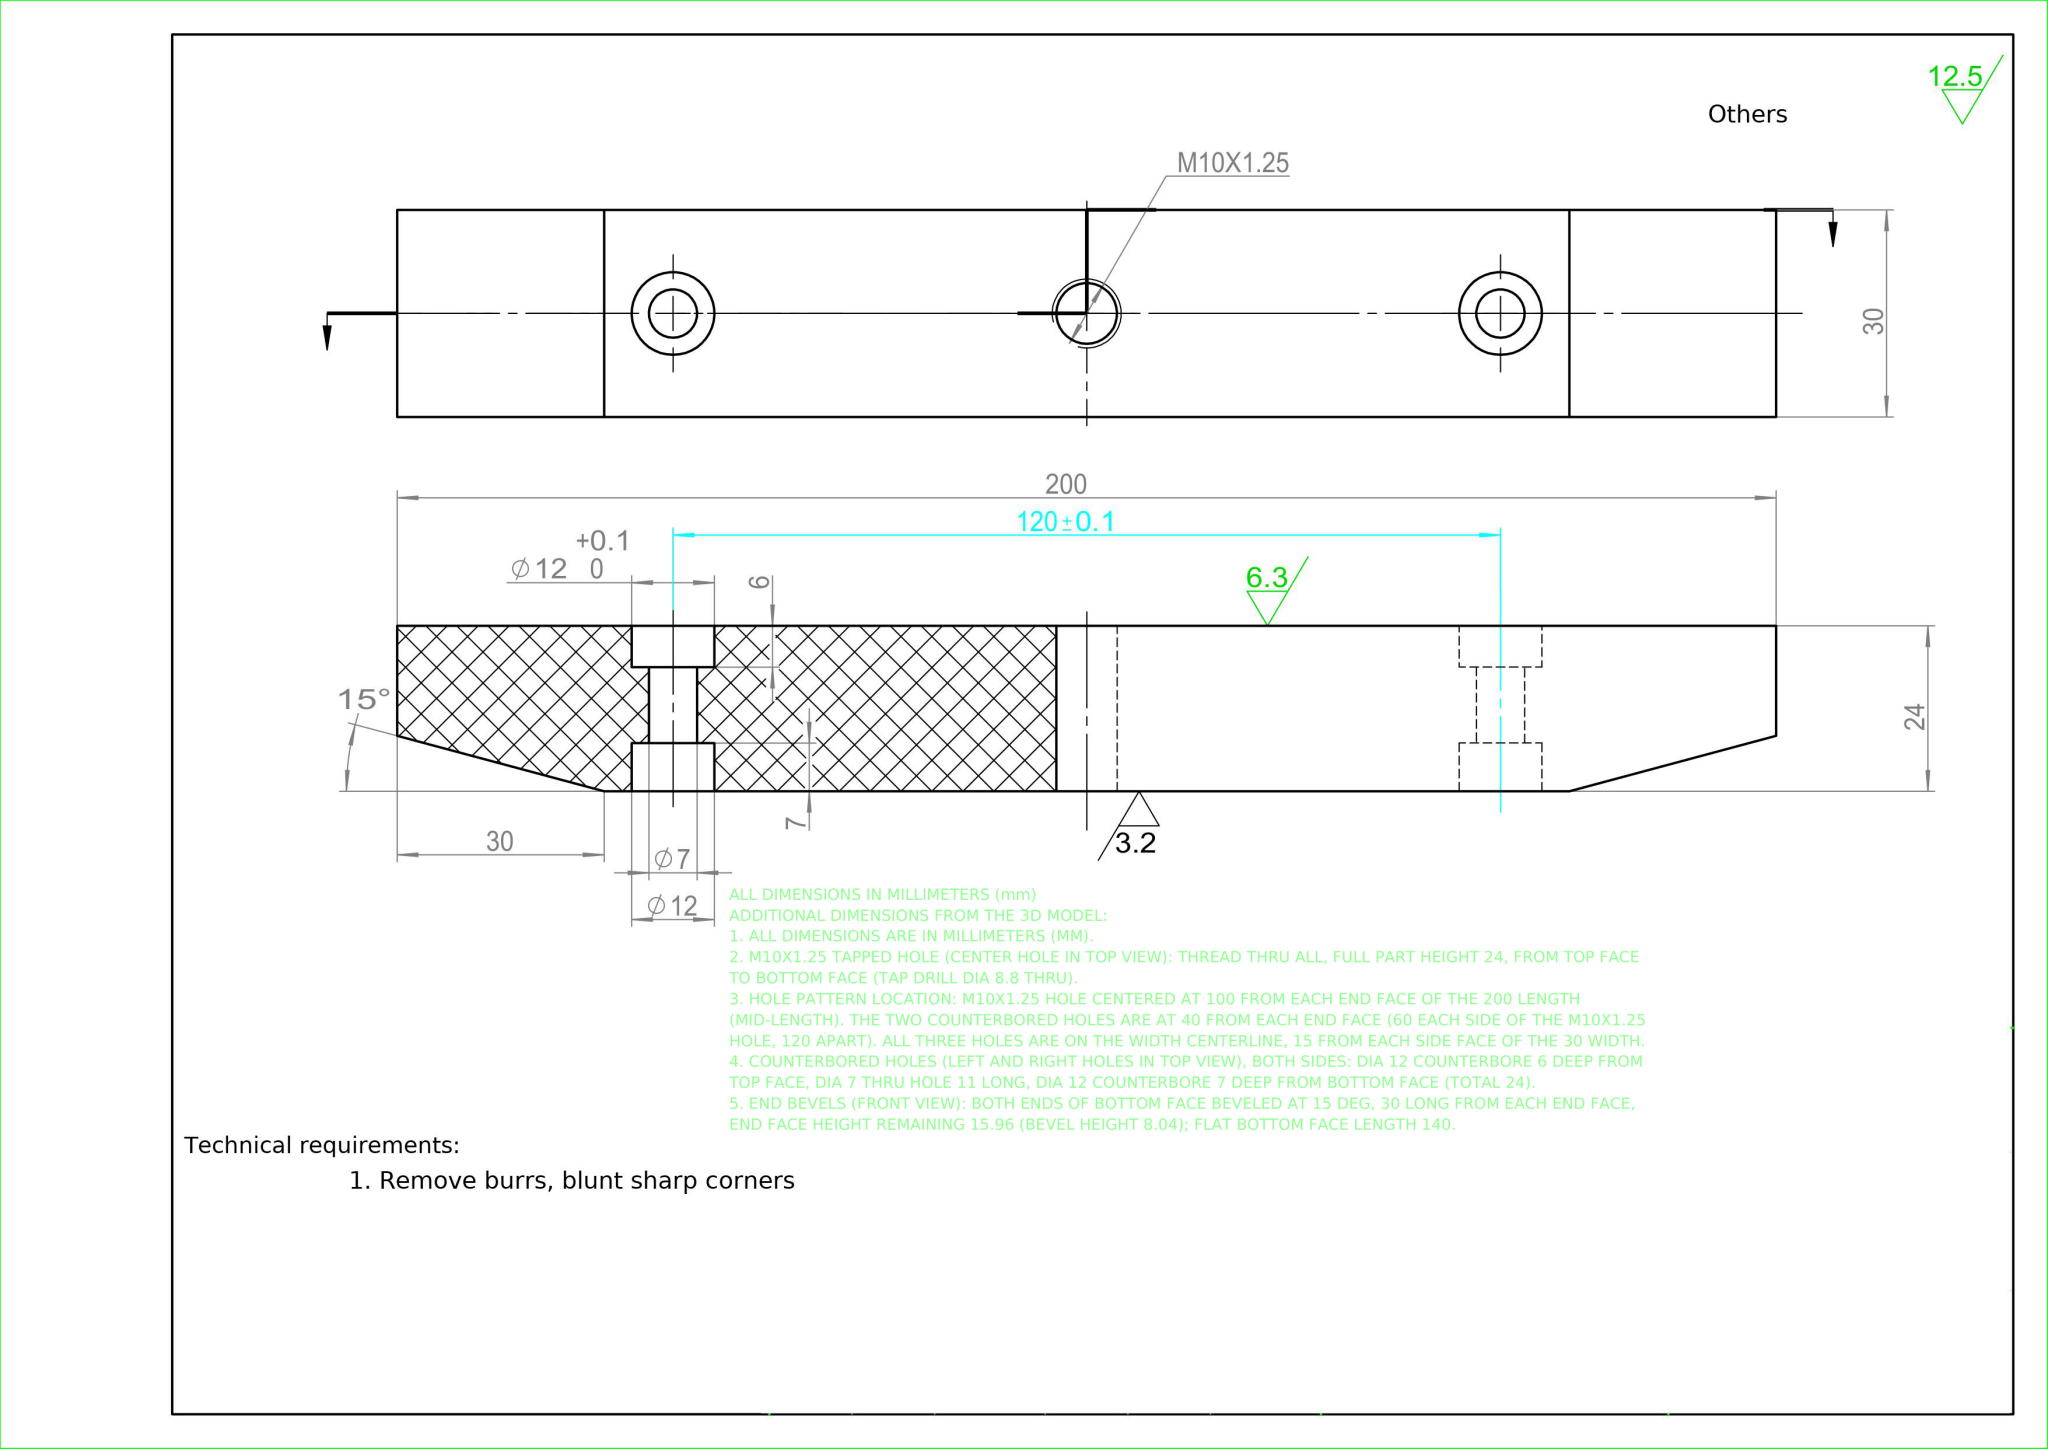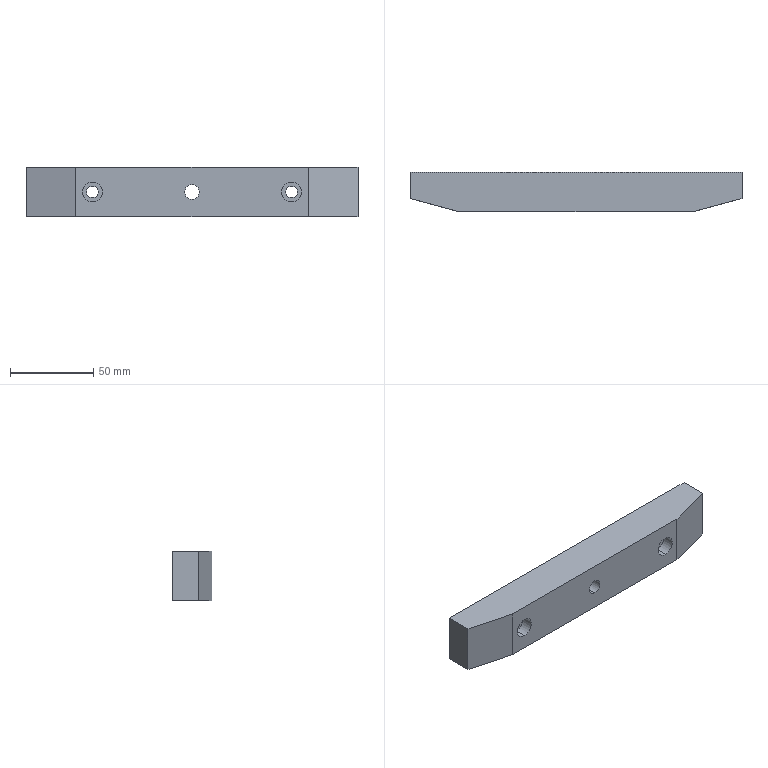Part | NX | mm | Tapered Threaded Mounting Bar | 1 solid | 26 faces | box 200 x 24 x 30 mm | volume 131518 mm3 | cylinder 14 | plane 12 | commonest cylinder face diameters 12 x8 7 x4 8.8 x2
STEP:
#1=COLOUR_RGB('',1.,1.,0.);
#2=FILL_AREA_STYLE_COLOUR('',#1);
#3=FILL_AREA_STYLE('',(#2));
#4=SURFACE_STYLE_FILL_AREA(#3);
#5=SURFACE_SIDE_STYLE('',(#4));
#6=SURFACE_STYLE_USAGE(.BOTH.,#5);
#7=PRESENTATION_STYLE_ASSIGNMENT((#6));
#8=CARTESIAN_POINT('',(66.,18.,15.));
#9=VERTEX_POINT('',#8);
#10=CARTESIAN_POINT('',(54.,18.,15.));
#11=VERTEX_POINT('',#10);
#12=CARTESIAN_POINT('',(60.,18.,15.));
#13=DIRECTION('',(-0.,1.,0.));
#14=DIRECTION('',(-1.,0.,0.));
#15=AXIS2_PLACEMENT_3D('',#12,#13,#14);
#16=CIRCLE('',#15,6.);
#17=EDGE_CURVE('',#9,#11,#16,.T.);
#18=ORIENTED_EDGE('',*,*,#17,.F.);
#19=CARTESIAN_POINT('',(66.,24.,15.));
#20=VERTEX_POINT('',#19);
#21=CARTESIAN_POINT('',(66.,18.,15.));
#22=DIRECTION('',(-0.,1.,0.));
#23=VECTOR('',#22,1000.);
#24=LINE('',#21,#23);
#25=EDGE_CURVE('',#9,#20,#24,.T.);
#26=ORIENTED_EDGE('',*,*,#25,.T.);
#27=CARTESIAN_POINT('',(54.,24.,15.));
#28=VERTEX_POINT('',#27);
#29=CARTESIAN_POINT('',(60.,24.,15.));
#30=DIRECTION('',(-0.,1.,0.));
#31=DIRECTION('',(-1.,0.,0.));
#32=AXIS2_PLACEMENT_3D('',#29,#30,#31);
#33=CIRCLE('',#32,6.);
#34=EDGE_CURVE('',#20,#28,#33,.T.);
#35=ORIENTED_EDGE('',*,*,#34,.T.);
#36=CARTESIAN_POINT('',(54.,18.,15.));
#37=DIRECTION('',(-0.,1.,0.));
#38=VECTOR('',#37,1000.);
#39=LINE('',#36,#38);
#40=EDGE_CURVE('',#11,#28,#39,.T.);
#41=ORIENTED_EDGE('',*,*,#40,.F.);
#42=EDGE_LOOP('',(#18,#26,#35,#41));
#43=FACE_OUTER_BOUND('',#42,.T.);
#44=CARTESIAN_POINT('',(60.,18.,15.));
#45=DIRECTION('',(-0.,1.,0.));
#46=DIRECTION('',(-1.,0.,0.));
#47=AXIS2_PLACEMENT_3D('',#44,#45,#46);
#48=CYLINDRICAL_SURFACE('',#47,6.);
#49=ADVANCED_FACE('',(#43),#48,.F.);
#50=CARTESIAN_POINT('',(-54.,18.,15.));
#51=VERTEX_POINT('',#50);
#52=CARTESIAN_POINT('',(-66.,18.,15.));
#53=VERTEX_POINT('',#52);
#54=CARTESIAN_POINT('',(-60.,18.,15.));
#55=DIRECTION('',(-0.,1.,0.));
#56=DIRECTION('',(-1.,0.,0.));
#57=AXIS2_PLACEMENT_3D('',#54,#55,#56);
#58=CIRCLE('',#57,6.);
#59=EDGE_CURVE('',#51,#53,#58,.T.);
#60=ORIENTED_EDGE('',*,*,#59,.F.);
#61=CARTESIAN_POINT('',(-54.,24.,15.));
#62=VERTEX_POINT('',#61);
#63=CARTESIAN_POINT('',(-54.,18.,15.));
#64=DIRECTION('',(-0.,1.,0.));
#65=VECTOR('',#64,1000.);
#66=LINE('',#63,#65);
#67=EDGE_CURVE('',#51,#62,#66,.T.);
#68=ORIENTED_EDGE('',*,*,#67,.T.);
#69=CARTESIAN_POINT('',(-66.,24.,15.));
#70=VERTEX_POINT('',#69);
#71=CARTESIAN_POINT('',(-60.,24.,15.));
#72=DIRECTION('',(-0.,1.,0.));
#73=DIRECTION('',(-1.,0.,0.));
#74=AXIS2_PLACEMENT_3D('',#71,#72,#73);
#75=CIRCLE('',#74,6.);
#76=EDGE_CURVE('',#62,#70,#75,.T.);
#77=ORIENTED_EDGE('',*,*,#76,.T.);
#78=CARTESIAN_POINT('',(-66.,18.,15.));
#79=DIRECTION('',(-0.,1.,0.));
#80=VECTOR('',#79,1000.);
#81=LINE('',#78,#80);
#82=EDGE_CURVE('',#53,#70,#81,.T.);
#83=ORIENTED_EDGE('',*,*,#82,.F.);
#84=EDGE_LOOP('',(#60,#68,#77,#83));
#85=FACE_OUTER_BOUND('',#84,.T.);
#86=CARTESIAN_POINT('',(-60.,18.,15.));
#87=DIRECTION('',(-0.,1.,0.));
#88=DIRECTION('',(-1.,0.,0.));
#89=AXIS2_PLACEMENT_3D('',#86,#87,#88);
#90=CYLINDRICAL_SURFACE('',#89,6.);
#91=ADVANCED_FACE('',(#85),#90,.F.);
#92=CARTESIAN_POINT('',(-60.,7.,21.));
#93=VERTEX_POINT('',#92);
#94=CARTESIAN_POINT('',(-60.,7.,9.));
#95=VERTEX_POINT('',#94);
#96=CARTESIAN_POINT('',(-60.,7.,15.));
#97=DIRECTION('',(0.,-1.,0.));
#98=DIRECTION('',(0.,0.,-1.));
#99=AXIS2_PLACEMENT_3D('',#96,#97,#98);
#100=CIRCLE('',#99,6.);
#101=EDGE_CURVE('',#93,#95,#100,.T.);
#102=ORIENTED_EDGE('',*,*,#101,.F.);
#103=CARTESIAN_POINT('',(-60.,-0.,21.));
#104=VERTEX_POINT('',#103);
#105=CARTESIAN_POINT('',(-60.,-0.,21.));
#106=DIRECTION('',(0.,-1.,0.));
#107=VECTOR('',#106,1000.);
#108=LINE('',#105,#107);
#109=EDGE_CURVE('',#93,#104,#108,.T.);
#110=ORIENTED_EDGE('',*,*,#109,.T.);
#111=CARTESIAN_POINT('',(-60.,-0.,9.));
#112=VERTEX_POINT('',#111);
#113=CARTESIAN_POINT('',(-60.,-0.,15.));
#114=DIRECTION('',(0.,-1.,0.));
#115=DIRECTION('',(0.,0.,-1.));
#116=AXIS2_PLACEMENT_3D('',#113,#114,#115);
#117=CIRCLE('',#116,6.);
#118=EDGE_CURVE('',#104,#112,#117,.T.);
#119=ORIENTED_EDGE('',*,*,#118,.T.);
#120=CARTESIAN_POINT('',(-60.,-0.,9.));
#121=DIRECTION('',(0.,-1.,0.));
#122=VECTOR('',#121,1000.);
#123=LINE('',#120,#122);
#124=EDGE_CURVE('',#95,#112,#123,.T.);
#125=ORIENTED_EDGE('',*,*,#124,.F.);
#126=EDGE_LOOP('',(#102,#110,#119,#125));
#127=FACE_OUTER_BOUND('',#126,.T.);
#128=CARTESIAN_POINT('',(-60.,-0.,15.));
#129=DIRECTION('',(0.,-1.,0.));
#130=DIRECTION('',(0.,0.,-1.));
#131=AXIS2_PLACEMENT_3D('',#128,#129,#130);
#132=CYLINDRICAL_SURFACE('',#131,6.);
#133=ADVANCED_FACE('',(#127),#132,.F.);
#134=CARTESIAN_POINT('',(60.,7.,21.));
#135=VERTEX_POINT('',#134);
#136=CARTESIAN_POINT('',(60.,7.,9.));
#137=VERTEX_POINT('',#136);
#138=CARTESIAN_POINT('',(60.,7.,15.));
#139=DIRECTION('',(0.,-1.,0.));
#140=DIRECTION('',(0.,0.,-1.));
#141=AXIS2_PLACEMENT_3D('',#138,#139,#140);
#142=CIRCLE('',#141,6.);
#143=EDGE_CURVE('',#135,#137,#142,.T.);
#144=ORIENTED_EDGE('',*,*,#143,.F.);
#145=CARTESIAN_POINT('',(60.,0.,21.));
#146=VERTEX_POINT('',#145);
#147=CARTESIAN_POINT('',(60.,0.,21.));
#148=DIRECTION('',(0.,-1.,0.));
#149=VECTOR('',#148,1000.);
#150=LINE('',#147,#149);
#151=EDGE_CURVE('',#135,#146,#150,.T.);
#152=ORIENTED_EDGE('',*,*,#151,.T.);
#153=CARTESIAN_POINT('',(60.,0.,9.));
#154=VERTEX_POINT('',#153);
#155=CARTESIAN_POINT('',(60.,0.,15.));
#156=DIRECTION('',(0.,-1.,0.));
#157=DIRECTION('',(0.,0.,-1.));
#158=AXIS2_PLACEMENT_3D('',#155,#156,#157);
#159=CIRCLE('',#158,6.);
#160=EDGE_CURVE('',#146,#154,#159,.T.);
#161=ORIENTED_EDGE('',*,*,#160,.T.);
#162=CARTESIAN_POINT('',(60.,0.,9.));
#163=DIRECTION('',(0.,-1.,0.));
#164=VECTOR('',#163,1000.);
#165=LINE('',#162,#164);
#166=EDGE_CURVE('',#137,#154,#165,.T.);
#167=ORIENTED_EDGE('',*,*,#166,.F.);
#168=EDGE_LOOP('',(#144,#152,#161,#167));
#169=FACE_OUTER_BOUND('',#168,.T.);
#170=CARTESIAN_POINT('',(60.,0.,15.));
#171=DIRECTION('',(0.,-1.,0.));
#172=DIRECTION('',(0.,0.,-1.));
#173=AXIS2_PLACEMENT_3D('',#170,#171,#172);
#174=CYLINDRICAL_SURFACE('',#173,6.);
#175=ADVANCED_FACE('',(#169),#174,.F.);
#176=CARTESIAN_POINT('',(0.,24.,19.4));
#177=VERTEX_POINT('',#176);
#178=CARTESIAN_POINT('',(0.,24.,10.6));
#179=VERTEX_POINT('',#178);
#180=CARTESIAN_POINT('',(0.,24.,15.));
#181=DIRECTION('',(0.,-1.,0.));
#182=DIRECTION('',(0.,0.,-1.));
#183=AXIS2_PLACEMENT_3D('',#180,#181,#182);
#184=CIRCLE('',#183,4.4);
#185=EDGE_CURVE('',#177,#179,#184,.T.);
#186=ORIENTED_EDGE('',*,*,#185,.F.);
#187=CARTESIAN_POINT('',(0.,-0.,19.4));
#188=VERTEX_POINT('',#187);
#189=CARTESIAN_POINT('',(0.,0.,19.4));
#190=DIRECTION('',(0.,-1.,0.));
#191=VECTOR('',#190,1000.);
#192=LINE('',#189,#191);
#193=EDGE_CURVE('',#177,#188,#192,.T.);
#194=ORIENTED_EDGE('',*,*,#193,.T.);
#195=CARTESIAN_POINT('',(0.,-0.,10.6));
#196=VERTEX_POINT('',#195);
#197=CARTESIAN_POINT('',(0.,-0.,15.));
#198=DIRECTION('',(0.,-1.,0.));
#199=DIRECTION('',(0.,0.,-1.));
#200=AXIS2_PLACEMENT_3D('',#197,#198,#199);
#201=CIRCLE('',#200,4.4);
#202=EDGE_CURVE('',#188,#196,#201,.T.);
#203=ORIENTED_EDGE('',*,*,#202,.T.);
#204=CARTESIAN_POINT('',(0.,0.,10.6));
#205=DIRECTION('',(0.,-1.,0.));
#206=VECTOR('',#205,1000.);
#207=LINE('',#204,#206);
#208=EDGE_CURVE('',#179,#196,#207,.T.);
#209=ORIENTED_EDGE('',*,*,#208,.F.);
#210=EDGE_LOOP('',(#186,#194,#203,#209));
#211=FACE_OUTER_BOUND('',#210,.T.);
#212=CARTESIAN_POINT('',(0.,0.,15.));
#213=DIRECTION('',(0.,-1.,0.));
#214=DIRECTION('',(0.,0.,-1.));
#215=AXIS2_PLACEMENT_3D('',#212,#213,#214);
#216=CYLINDRICAL_SURFACE('',#215,4.4);
#217=ADVANCED_FACE('',(#211),#216,.F.);
#218=CARTESIAN_POINT('',(-60.,18.,18.5));
#219=VERTEX_POINT('',#218);
#220=CARTESIAN_POINT('',(-60.,18.,11.5));
#221=VERTEX_POINT('',#220);
#222=CARTESIAN_POINT('',(-60.,18.,15.));
#223=DIRECTION('',(0.,-1.,0.));
#224=DIRECTION('',(-1.,0.,0.));
#225=AXIS2_PLACEMENT_3D('',#222,#223,#224);
#226=CIRCLE('',#225,3.5);
#227=EDGE_CURVE('',#219,#221,#226,.T.);
#228=ORIENTED_EDGE('',*,*,#227,.F.);
#229=CARTESIAN_POINT('',(-60.,7.,18.5));
#230=VERTEX_POINT('',#229);
#231=CARTESIAN_POINT('',(-60.,-0.,18.5));
#232=DIRECTION('',(0.,-1.,0.));
#233=VECTOR('',#232,1000.);
#234=LINE('',#231,#233);
#235=EDGE_CURVE('',#219,#230,#234,.T.);
#236=ORIENTED_EDGE('',*,*,#235,.T.);
#237=CARTESIAN_POINT('',(-60.,7.,11.5));
#238=VERTEX_POINT('',#237);
#239=CARTESIAN_POINT('',(-60.,7.,15.));
#240=DIRECTION('',(0.,-1.,0.));
#241=DIRECTION('',(0.,0.,-1.));
#242=AXIS2_PLACEMENT_3D('',#239,#240,#241);
#243=CIRCLE('',#242,3.5);
#244=EDGE_CURVE('',#230,#238,#243,.T.);
#245=ORIENTED_EDGE('',*,*,#244,.T.);
#246=CARTESIAN_POINT('',(-60.,-0.,11.5));
#247=DIRECTION('',(0.,-1.,0.));
#248=VECTOR('',#247,1000.);
#249=LINE('',#246,#248);
#250=EDGE_CURVE('',#221,#238,#249,.T.);
#251=ORIENTED_EDGE('',*,*,#250,.F.);
#252=EDGE_LOOP('',(#228,#236,#245,#251));
#253=FACE_OUTER_BOUND('',#252,.T.);
#254=CARTESIAN_POINT('',(-60.,-0.,15.));
#255=DIRECTION('',(0.,-1.,0.));
#256=DIRECTION('',(0.,0.,-1.));
#257=AXIS2_PLACEMENT_3D('',#254,#255,#256);
#258=CYLINDRICAL_SURFACE('',#257,3.5);
#259=ADVANCED_FACE('',(#253),#258,.F.);
#260=CARTESIAN_POINT('',(60.,18.,18.5));
#261=VERTEX_POINT('',#260);
#262=CARTESIAN_POINT('',(60.,18.,11.5));
#263=VERTEX_POINT('',#262);
#264=CARTESIAN_POINT('',(60.,18.,15.));
#265=DIRECTION('',(0.,-1.,0.));
#266=DIRECTION('',(-1.,0.,0.));
#267=AXIS2_PLACEMENT_3D('',#264,#265,#266);
#268=CIRCLE('',#267,3.5);
#269=EDGE_CURVE('',#261,#263,#268,.T.);
#270=ORIENTED_EDGE('',*,*,#269,.F.);
#271=CARTESIAN_POINT('',(60.,7.,18.5));
#272=VERTEX_POINT('',#271);
#273=CARTESIAN_POINT('',(60.,0.,18.5));
#274=DIRECTION('',(0.,-1.,0.));
#275=VECTOR('',#274,1000.);
#276=LINE('',#273,#275);
#277=EDGE_CURVE('',#261,#272,#276,.T.);
#278=ORIENTED_EDGE('',*,*,#277,.T.);
#279=CARTESIAN_POINT('',(60.,7.,11.5));
#280=VERTEX_POINT('',#279);
#281=CARTESIAN_POINT('',(60.,7.,15.));
#282=DIRECTION('',(0.,-1.,0.));
#283=DIRECTION('',(0.,0.,-1.));
#284=AXIS2_PLACEMENT_3D('',#281,#282,#283);
#285=CIRCLE('',#284,3.5);
#286=EDGE_CURVE('',#272,#280,#285,.T.);
#287=ORIENTED_EDGE('',*,*,#286,.T.);
#288=CARTESIAN_POINT('',(60.,0.,11.5));
#289=DIRECTION('',(0.,-1.,0.));
#290=VECTOR('',#289,1000.);
#291=LINE('',#288,#290);
#292=EDGE_CURVE('',#263,#280,#291,.T.);
#293=ORIENTED_EDGE('',*,*,#292,.F.);
#294=EDGE_LOOP('',(#270,#278,#287,#293));
#295=FACE_OUTER_BOUND('',#294,.T.);
#296=CARTESIAN_POINT('',(60.,0.,15.));
#297=DIRECTION('',(0.,-1.,0.));
#298=DIRECTION('',(0.,0.,-1.));
#299=AXIS2_PLACEMENT_3D('',#296,#297,#298);
#300=CYLINDRICAL_SURFACE('',#299,3.5);
#301=ADVANCED_FACE('',(#295),#300,.F.);
#302=ORIENTED_EDGE('',*,*,#277,.F.);
#303=CARTESIAN_POINT('',(60.,18.,15.));
#304=DIRECTION('',(0.,-1.,0.));
#305=DIRECTION('',(-1.,0.,0.));
#306=AXIS2_PLACEMENT_3D('',#303,#304,#305);
#307=CIRCLE('',#306,3.5);
#308=EDGE_CURVE('',#263,#261,#307,.T.);
#309=ORIENTED_EDGE('',*,*,#308,.F.);
#310=ORIENTED_EDGE('',*,*,#292,.T.);
#311=CARTESIAN_POINT('',(60.,7.,15.));
#312=DIRECTION('',(0.,-1.,0.));
#313=DIRECTION('',(0.,0.,-1.));
#314=AXIS2_PLACEMENT_3D('',#311,#312,#313);
#315=CIRCLE('',#314,3.5);
#316=EDGE_CURVE('',#280,#272,#315,.T.);
#317=ORIENTED_EDGE('',*,*,#316,.T.);
#318=EDGE_LOOP('',(#302,#309,#310,#317));
#319=FACE_OUTER_BOUND('',#318,.T.);
#320=CARTESIAN_POINT('',(60.,0.,15.));
#321=DIRECTION('',(0.,-1.,0.));
#322=DIRECTION('',(0.,0.,-1.));
#323=AXIS2_PLACEMENT_3D('',#320,#321,#322);
#324=CYLINDRICAL_SURFACE('',#323,3.5);
#325=ADVANCED_FACE('',(#319),#324,.F.);
#326=ORIENTED_EDGE('',*,*,#235,.F.);
#327=CARTESIAN_POINT('',(-60.,18.,15.));
#328=DIRECTION('',(0.,-1.,0.));
#329=DIRECTION('',(-1.,0.,0.));
#330=AXIS2_PLACEMENT_3D('',#327,#328,#329);
#331=CIRCLE('',#330,3.5);
#332=EDGE_CURVE('',#221,#219,#331,.T.);
#333=ORIENTED_EDGE('',*,*,#332,.F.);
#334=ORIENTED_EDGE('',*,*,#250,.T.);
#335=CARTESIAN_POINT('',(-60.,7.,15.));
#336=DIRECTION('',(0.,-1.,0.));
#337=DIRECTION('',(0.,0.,-1.));
#338=AXIS2_PLACEMENT_3D('',#335,#336,#337);
#339=CIRCLE('',#338,3.5);
#340=EDGE_CURVE('',#238,#230,#339,.T.);
#341=ORIENTED_EDGE('',*,*,#340,.T.);
#342=EDGE_LOOP('',(#326,#333,#334,#341));
#343=FACE_OUTER_BOUND('',#342,.T.);
#344=CARTESIAN_POINT('',(-60.,-0.,15.));
#345=DIRECTION('',(0.,-1.,0.));
#346=DIRECTION('',(0.,0.,-1.));
#347=AXIS2_PLACEMENT_3D('',#344,#345,#346);
#348=CYLINDRICAL_SURFACE('',#347,3.5);
#349=ADVANCED_FACE('',(#343),#348,.F.);
#350=CARTESIAN_POINT('',(70.,-0.,0.));
#351=VERTEX_POINT('',#350);
#352=CARTESIAN_POINT('',(100.,8.038,0.));
#353=VERTEX_POINT('',#352);
#354=CARTESIAN_POINT('',(100.,8.038,0.));
#355=DIRECTION('',(0.9659,0.2588,0.));
#356=VECTOR('',#355,1000.);
#357=LINE('',#354,#356);
#358=EDGE_CURVE('',#351,#353,#357,.T.);
#359=ORIENTED_EDGE('',*,*,#358,.T.);
#360=CARTESIAN_POINT('',(100.,8.038,30.));
#361=VERTEX_POINT('',#360);
#362=CARTESIAN_POINT('',(100.,8.038,30.));
#363=DIRECTION('',(0.,0.,-1.));
#364=VECTOR('',#363,1000.);
#365=LINE('',#362,#364);
#366=EDGE_CURVE('',#361,#353,#365,.T.);
#367=ORIENTED_EDGE('',*,*,#366,.F.);
#368=CARTESIAN_POINT('',(70.,-0.,30.));
#369=VERTEX_POINT('',#368);
#370=CARTESIAN_POINT('',(100.,8.038,30.));
#371=DIRECTION('',(0.9659,0.2588,0.));
#372=VECTOR('',#371,1000.);
#373=LINE('',#370,#372);
#374=EDGE_CURVE('',#369,#361,#373,.T.);
#375=ORIENTED_EDGE('',*,*,#374,.F.);
#376=CARTESIAN_POINT('',(70.,-0.,30.));
#377=DIRECTION('',(0.,0.,-1.));
#378=VECTOR('',#377,1000.);
#379=LINE('',#376,#378);
#380=EDGE_CURVE('',#369,#351,#379,.T.);
#381=ORIENTED_EDGE('',*,*,#380,.T.);
#382=EDGE_LOOP('',(#359,#367,#375,#381));
#383=FACE_OUTER_BOUND('',#382,.T.);
#384=CARTESIAN_POINT('',(100.,8.038,30.));
#385=DIRECTION('',(-0.2588,0.9659,0.));
#386=DIRECTION('',(-0.9659,-0.2588,0.));
#387=AXIS2_PLACEMENT_3D('',#384,#385,#386);
#388=PLANE('',#387);
#389=ADVANCED_FACE('',(#383),#388,.F.);
#390=CARTESIAN_POINT('',(100.,24.,0.));
#391=VERTEX_POINT('',#390);
#392=CARTESIAN_POINT('',(100.,8.038,0.));
#393=DIRECTION('',(0.,1.,0.));
#394=VECTOR('',#393,1000.);
#395=LINE('',#392,#394);
#396=EDGE_CURVE('',#353,#391,#395,.T.);
#397=ORIENTED_EDGE('',*,*,#396,.T.);
#398=CARTESIAN_POINT('',(100.,24.,30.));
#399=VERTEX_POINT('',#398);
#400=CARTESIAN_POINT('',(100.,24.,30.));
#401=DIRECTION('',(0.,0.,-1.));
#402=VECTOR('',#401,1000.);
#403=LINE('',#400,#402);
#404=EDGE_CURVE('',#399,#391,#403,.T.);
#405=ORIENTED_EDGE('',*,*,#404,.F.);
#406=CARTESIAN_POINT('',(100.,8.038,30.));
#407=DIRECTION('',(0.,1.,0.));
#408=VECTOR('',#407,1000.);
#409=LINE('',#406,#408);
#410=EDGE_CURVE('',#361,#399,#409,.T.);
#411=ORIENTED_EDGE('',*,*,#410,.F.);
#412=ORIENTED_EDGE('',*,*,#366,.T.);
#413=EDGE_LOOP('',(#397,#405,#411,#412));
#414=FACE_OUTER_BOUND('',#413,.T.);
#415=CARTESIAN_POINT('',(100.,8.038,30.));
#416=DIRECTION('',(-1.,0.,0.));
#417=DIRECTION('',(0.,0.,1.));
#418=AXIS2_PLACEMENT_3D('',#415,#416,#417);
#419=PLANE('',#418);
#420=ADVANCED_FACE('',(#414),#419,.F.);
#421=CARTESIAN_POINT('',(60.,24.,15.));
#422=DIRECTION('',(-0.,1.,0.));
#423=DIRECTION('',(-1.,0.,0.));
#424=AXIS2_PLACEMENT_3D('',#421,#422,#423);
#425=CIRCLE('',#424,6.);
#426=EDGE_CURVE('',#28,#20,#425,.T.);
#427=ORIENTED_EDGE('',*,*,#426,.F.);
#428=ORIENTED_EDGE('',*,*,#34,.F.);
#429=EDGE_LOOP('',(#427,#428));
#430=FACE_BOUND('',#429,.T.);
#431=CARTESIAN_POINT('',(-60.,24.,15.));
#432=DIRECTION('',(-0.,1.,0.));
#433=DIRECTION('',(-1.,0.,0.));
#434=AXIS2_PLACEMENT_3D('',#431,#432,#433);
#435=CIRCLE('',#434,6.);
#436=EDGE_CURVE('',#70,#62,#435,.T.);
#437=ORIENTED_EDGE('',*,*,#436,.F.);
#438=ORIENTED_EDGE('',*,*,#76,.F.);
#439=EDGE_LOOP('',(#437,#438));
#440=FACE_BOUND('',#439,.T.);
#441=CARTESIAN_POINT('',(0.,24.,15.));
#442=DIRECTION('',(0.,-1.,0.));
#443=DIRECTION('',(0.,0.,-1.));
#444=AXIS2_PLACEMENT_3D('',#441,#442,#443);
#445=CIRCLE('',#444,4.4);
#446=EDGE_CURVE('',#179,#177,#445,.T.);
#447=ORIENTED_EDGE('',*,*,#446,.T.);
#448=ORIENTED_EDGE('',*,*,#185,.T.);
#449=EDGE_LOOP('',(#447,#448));
#450=FACE_BOUND('',#449,.T.);
#451=CARTESIAN_POINT('',(-100.,24.,0.));
#452=VERTEX_POINT('',#451);
#453=CARTESIAN_POINT('',(-100.,24.,0.));
#454=DIRECTION('',(-1.,-0.,0.));
#455=VECTOR('',#454,1000.);
#456=LINE('',#453,#455);
#457=EDGE_CURVE('',#391,#452,#456,.T.);
#458=ORIENTED_EDGE('',*,*,#457,.T.);
#459=CARTESIAN_POINT('',(-100.,24.,30.));
#460=VERTEX_POINT('',#459);
#461=CARTESIAN_POINT('',(-100.,24.,30.));
#462=DIRECTION('',(0.,0.,-1.));
#463=VECTOR('',#462,1000.);
#464=LINE('',#461,#463);
#465=EDGE_CURVE('',#460,#452,#464,.T.);
#466=ORIENTED_EDGE('',*,*,#465,.F.);
#467=CARTESIAN_POINT('',(-100.,24.,30.));
#468=DIRECTION('',(-1.,-0.,0.));
#469=VECTOR('',#468,1000.);
#470=LINE('',#467,#469);
#471=EDGE_CURVE('',#399,#460,#470,.T.);
#472=ORIENTED_EDGE('',*,*,#471,.F.);
#473=ORIENTED_EDGE('',*,*,#404,.T.);
#474=EDGE_LOOP('',(#458,#466,#472,#473));
#475=FACE_OUTER_BOUND('',#474,.T.);
#476=CARTESIAN_POINT('',(-100.,24.,30.));
#477=DIRECTION('',(0.,-1.,0.));
#478=DIRECTION('',(1.,0.,0.));
#479=AXIS2_PLACEMENT_3D('',#476,#477,#478);
#480=PLANE('',#479);
#481=ADVANCED_FACE('',(#430,#440,#450,#475),#480,.F.);
#482=CARTESIAN_POINT('',(-100.,8.038,0.));
#483=VERTEX_POINT('',#482);
#484=CARTESIAN_POINT('',(-100.,8.038,0.));
#485=DIRECTION('',(0.,-1.,0.));
#486=VECTOR('',#485,1000.);
#487=LINE('',#484,#486);
#488=EDGE_CURVE('',#452,#483,#487,.T.);
#489=ORIENTED_EDGE('',*,*,#488,.T.);
#490=CARTESIAN_POINT('',(-100.,8.038,30.));
#491=VERTEX_POINT('',#490);
#492=CARTESIAN_POINT('',(-100.,8.038,30.));
#493=DIRECTION('',(0.,0.,-1.));
#494=VECTOR('',#493,1000.);
#495=LINE('',#492,#494);
#496=EDGE_CURVE('',#491,#483,#495,.T.);
#497=ORIENTED_EDGE('',*,*,#496,.F.);
#498=CARTESIAN_POINT('',(-100.,8.038,30.));
#499=DIRECTION('',(0.,-1.,0.));
#500=VECTOR('',#499,1000.);
#501=LINE('',#498,#500);
#502=EDGE_CURVE('',#460,#491,#501,.T.);
#503=ORIENTED_EDGE('',*,*,#502,.F.);
#504=ORIENTED_EDGE('',*,*,#465,.T.);
#505=EDGE_LOOP('',(#489,#497,#503,#504));
#506=FACE_OUTER_BOUND('',#505,.T.);
#507=CARTESIAN_POINT('',(-100.,8.038,30.));
#508=DIRECTION('',(1.,0.,0.));
#509=DIRECTION('',(0.,0.,-1.));
#510=AXIS2_PLACEMENT_3D('',#507,#508,#509);
#511=PLANE('',#510);
#512=ADVANCED_FACE('',(#506),#511,.F.);
#513=CARTESIAN_POINT('',(-70.,-0.,0.));
#514=VERTEX_POINT('',#513);
#515=CARTESIAN_POINT('',(-100.,8.038,0.));
#516=DIRECTION('',(0.9659,-0.2588,0.));
#517=VECTOR('',#516,1000.);
#518=LINE('',#515,#517);
#519=EDGE_CURVE('',#483,#514,#518,.T.);
#520=ORIENTED_EDGE('',*,*,#519,.T.);
#521=CARTESIAN_POINT('',(-70.,-0.,30.));
#522=VERTEX_POINT('',#521);
#523=CARTESIAN_POINT('',(-70.,-0.,30.));
#524=DIRECTION('',(0.,0.,-1.));
#525=VECTOR('',#524,1000.);
#526=LINE('',#523,#525);
#527=EDGE_CURVE('',#522,#514,#526,.T.);
#528=ORIENTED_EDGE('',*,*,#527,.F.);
#529=CARTESIAN_POINT('',(-100.,8.038,30.));
#530=DIRECTION('',(0.9659,-0.2588,0.));
#531=VECTOR('',#530,1000.);
#532=LINE('',#529,#531);
#533=EDGE_CURVE('',#491,#522,#532,.T.);
#534=ORIENTED_EDGE('',*,*,#533,.F.);
#535=ORIENTED_EDGE('',*,*,#496,.T.);
#536=EDGE_LOOP('',(#520,#528,#534,#535));
#537=FACE_OUTER_BOUND('',#536,.T.);
#538=CARTESIAN_POINT('',(-100.,8.038,30.));
#539=DIRECTION('',(0.2588,0.9659,0.));
#540=DIRECTION('',(-0.9659,0.2588,0.));
#541=AXIS2_PLACEMENT_3D('',#538,#539,#540);
#542=PLANE('',#541);
#543=ADVANCED_FACE('',(#537),#542,.F.);
#544=CARTESIAN_POINT('',(-60.,-0.,15.));
#545=DIRECTION('',(0.,-1.,0.));
#546=DIRECTION('',(0.,0.,-1.));
#547=AXIS2_PLACEMENT_3D('',#544,#545,#546);
#548=CIRCLE('',#547,6.);
#549=EDGE_CURVE('',#112,#104,#548,.T.);
#550=ORIENTED_EDGE('',*,*,#549,.F.);
#551=ORIENTED_EDGE('',*,*,#118,.F.);
#552=EDGE_LOOP('',(#550,#551));
#553=FACE_BOUND('',#552,.T.);
#554=CARTESIAN_POINT('',(60.,0.,15.));
#555=DIRECTION('',(0.,-1.,0.));
#556=DIRECTION('',(0.,0.,-1.));
#557=AXIS2_PLACEMENT_3D('',#554,#555,#556);
#558=CIRCLE('',#557,6.);
#559=EDGE_CURVE('',#154,#146,#558,.T.);
#560=ORIENTED_EDGE('',*,*,#559,.F.);
#561=ORIENTED_EDGE('',*,*,#160,.F.);
#562=EDGE_LOOP('',(#560,#561));
#563=FACE_BOUND('',#562,.T.);
#564=CARTESIAN_POINT('',(0.,-0.,15.));
#565=DIRECTION('',(0.,-1.,0.));
#566=DIRECTION('',(0.,0.,-1.));
#567=AXIS2_PLACEMENT_3D('',#564,#565,#566);
#568=CIRCLE('',#567,4.4);
#569=EDGE_CURVE('',#196,#188,#568,.T.);
#570=ORIENTED_EDGE('',*,*,#569,.F.);
#571=ORIENTED_EDGE('',*,*,#202,.F.);
#572=EDGE_LOOP('',(#570,#571));
#573=FACE_BOUND('',#572,.T.);
#574=CARTESIAN_POINT('',(-70.,-0.,0.));
#575=DIRECTION('',(1.,0.,0.));
#576=VECTOR('',#575,1000.);
#577=LINE('',#574,#576);
#578=EDGE_CURVE('',#514,#351,#577,.T.);
#579=ORIENTED_EDGE('',*,*,#578,.T.);
#580=ORIENTED_EDGE('',*,*,#380,.F.);
#581=CARTESIAN_POINT('',(-70.,-0.,30.));
#582=DIRECTION('',(1.,0.,0.));
#583=VECTOR('',#582,1000.);
#584=LINE('',#581,#583);
#585=EDGE_CURVE('',#522,#369,#584,.T.);
#586=ORIENTED_EDGE('',*,*,#585,.F.);
#587=ORIENTED_EDGE('',*,*,#527,.T.);
#588=EDGE_LOOP('',(#579,#580,#586,#587));
#589=FACE_OUTER_BOUND('',#588,.T.);
#590=CARTESIAN_POINT('',(-70.,-0.,30.));
#591=DIRECTION('',(-0.,1.,0.));
#592=DIRECTION('',(-1.,-0.,0.));
#593=AXIS2_PLACEMENT_3D('',#590,#591,#592);
#594=PLANE('',#593);
#595=ADVANCED_FACE('',(#553,#563,#573,#589),#594,.F.);
#596=ORIENTED_EDGE('',*,*,#374,.T.);
#597=ORIENTED_EDGE('',*,*,#410,.T.);
#598=ORIENTED_EDGE('',*,*,#471,.T.);
#599=ORIENTED_EDGE('',*,*,#502,.T.);
#600=ORIENTED_EDGE('',*,*,#533,.T.);
#601=ORIENTED_EDGE('',*,*,#585,.T.);
#602=EDGE_LOOP('',(#596,#597,#598,#599,#600,#601));
#603=FACE_OUTER_BOUND('',#602,.T.);
#604=CARTESIAN_POINT('',(-100.,-45.551,30.));
#605=DIRECTION('',(0.,0.,-1.));
#606=DIRECTION('',(-1.,0.,0.));
#607=AXIS2_PLACEMENT_3D('',#604,#605,#606);
#608=PLANE('',#607);
#609=ADVANCED_FACE('',(#603),#608,.F.);
#610=ORIENTED_EDGE('',*,*,#358,.F.);
#611=ORIENTED_EDGE('',*,*,#578,.F.);
#612=ORIENTED_EDGE('',*,*,#519,.F.);
#613=ORIENTED_EDGE('',*,*,#488,.F.);
#614=ORIENTED_EDGE('',*,*,#457,.F.);
#615=ORIENTED_EDGE('',*,*,#396,.F.);
#616=EDGE_LOOP('',(#610,#611,#612,#613,#614,#615));
#617=FACE_OUTER_BOUND('',#616,.T.);
#618=CARTESIAN_POINT('',(-100.,-45.551,0.));
#619=DIRECTION('',(0.,0.,-1.));
#620=DIRECTION('',(-1.,0.,0.));
#621=AXIS2_PLACEMENT_3D('',#618,#619,#620);
#622=PLANE('',#621);
#623=ADVANCED_FACE('',(#617),#622,.T.);
#624=ORIENTED_EDGE('',*,*,#193,.F.);
#625=ORIENTED_EDGE('',*,*,#446,.F.);
#626=ORIENTED_EDGE('',*,*,#208,.T.);
#627=ORIENTED_EDGE('',*,*,#569,.T.);
#628=EDGE_LOOP('',(#624,#625,#626,#627));
#629=FACE_OUTER_BOUND('',#628,.T.);
#630=CARTESIAN_POINT('',(0.,0.,15.));
#631=DIRECTION('',(0.,-1.,0.));
#632=DIRECTION('',(0.,0.,-1.));
#633=AXIS2_PLACEMENT_3D('',#630,#631,#632);
#634=CYLINDRICAL_SURFACE('',#633,4.4);
#635=ADVANCED_FACE('',(#629),#634,.F.);
#636=ORIENTED_EDGE('',*,*,#316,.F.);
#637=ORIENTED_EDGE('',*,*,#286,.F.);
#638=EDGE_LOOP('',(#636,#637));
#639=FACE_BOUND('',#638,.T.);
#640=CARTESIAN_POINT('',(60.,7.,15.));
#641=DIRECTION('',(0.,-1.,0.));
#642=DIRECTION('',(0.,0.,-1.));
#643=AXIS2_PLACEMENT_3D('',#640,#641,#642);
#644=CIRCLE('',#643,6.);
#645=EDGE_CURVE('',#137,#135,#644,.T.);
#646=ORIENTED_EDGE('',*,*,#645,.T.);
#647=ORIENTED_EDGE('',*,*,#143,.T.);
#648=EDGE_LOOP('',(#646,#647));
#649=FACE_OUTER_BOUND('',#648,.T.);
#650=CARTESIAN_POINT('',(63.5,7.,15.));
#651=DIRECTION('',(0.,1.,0.));
#652=DIRECTION('',(0.,0.,1.));
#653=AXIS2_PLACEMENT_3D('',#650,#651,#652);
#654=PLANE('',#653);
#655=ADVANCED_FACE('',(#639,#649),#654,.F.);
#656=ORIENTED_EDGE('',*,*,#151,.F.);
#657=ORIENTED_EDGE('',*,*,#645,.F.);
#658=ORIENTED_EDGE('',*,*,#166,.T.);
#659=ORIENTED_EDGE('',*,*,#559,.T.);
#660=EDGE_LOOP('',(#656,#657,#658,#659));
#661=FACE_OUTER_BOUND('',#660,.T.);
#662=CARTESIAN_POINT('',(60.,0.,15.));
#663=DIRECTION('',(0.,-1.,0.));
#664=DIRECTION('',(0.,0.,-1.));
#665=AXIS2_PLACEMENT_3D('',#662,#663,#664);
#666=CYLINDRICAL_SURFACE('',#665,6.);
#667=ADVANCED_FACE('',(#661),#666,.F.);
#668=ORIENTED_EDGE('',*,*,#340,.F.);
#669=ORIENTED_EDGE('',*,*,#244,.F.);
#670=EDGE_LOOP('',(#668,#669));
#671=FACE_BOUND('',#670,.T.);
#672=CARTESIAN_POINT('',(-60.,7.,15.));
#673=DIRECTION('',(0.,-1.,0.));
#674=DIRECTION('',(0.,0.,-1.));
#675=AXIS2_PLACEMENT_3D('',#672,#673,#674);
#676=CIRCLE('',#675,6.);
#677=EDGE_CURVE('',#95,#93,#676,.T.);
#678=ORIENTED_EDGE('',*,*,#677,.T.);
#679=ORIENTED_EDGE('',*,*,#101,.T.);
#680=EDGE_LOOP('',(#678,#679));
#681=FACE_OUTER_BOUND('',#680,.T.);
#682=CARTESIAN_POINT('',(-56.5,7.,15.));
#683=DIRECTION('',(0.,1.,0.));
#684=DIRECTION('',(0.,0.,1.));
#685=AXIS2_PLACEMENT_3D('',#682,#683,#684);
#686=PLANE('',#685);
#687=ADVANCED_FACE('',(#671,#681),#686,.F.);
#688=ORIENTED_EDGE('',*,*,#109,.F.);
#689=ORIENTED_EDGE('',*,*,#677,.F.);
#690=ORIENTED_EDGE('',*,*,#124,.T.);
#691=ORIENTED_EDGE('',*,*,#549,.T.);
#692=EDGE_LOOP('',(#688,#689,#690,#691));
#693=FACE_OUTER_BOUND('',#692,.T.);
#694=CARTESIAN_POINT('',(-60.,-0.,15.));
#695=DIRECTION('',(0.,-1.,0.));
#696=DIRECTION('',(0.,0.,-1.));
#697=AXIS2_PLACEMENT_3D('',#694,#695,#696);
#698=CYLINDRICAL_SURFACE('',#697,6.);
#699=ADVANCED_FACE('',(#693),#698,.F.);
#700=CARTESIAN_POINT('',(-60.,18.,15.));
#701=DIRECTION('',(-0.,1.,0.));
#702=DIRECTION('',(-1.,0.,0.));
#703=AXIS2_PLACEMENT_3D('',#700,#701,#702);
#704=CIRCLE('',#703,6.);
#705=EDGE_CURVE('',#53,#51,#704,.T.);
#706=ORIENTED_EDGE('',*,*,#705,.T.);
#707=ORIENTED_EDGE('',*,*,#59,.T.);
#708=EDGE_LOOP('',(#706,#707));
#709=FACE_OUTER_BOUND('',#708,.T.);
#710=ORIENTED_EDGE('',*,*,#332,.T.);
#711=ORIENTED_EDGE('',*,*,#227,.T.);
#712=EDGE_LOOP('',(#710,#711));
#713=FACE_BOUND('',#712,.T.);
#714=CARTESIAN_POINT('',(-60.,18.,15.));
#715=DIRECTION('',(-0.,1.,0.));
#716=DIRECTION('',(-1.,-0.,0.));
#717=AXIS2_PLACEMENT_3D('',#714,#715,#716);
#718=PLANE('',#717);
#719=ADVANCED_FACE('',(#709,#713),#718,.T.);
#720=ORIENTED_EDGE('',*,*,#67,.F.);
#721=ORIENTED_EDGE('',*,*,#705,.F.);
#722=ORIENTED_EDGE('',*,*,#82,.T.);
#723=ORIENTED_EDGE('',*,*,#436,.T.);
#724=EDGE_LOOP('',(#720,#721,#722,#723));
#725=FACE_OUTER_BOUND('',#724,.T.);
#726=CARTESIAN_POINT('',(-60.,18.,15.));
#727=DIRECTION('',(-0.,1.,0.));
#728=DIRECTION('',(-1.,0.,0.));
#729=AXIS2_PLACEMENT_3D('',#726,#727,#728);
#730=CYLINDRICAL_SURFACE('',#729,6.);
#731=ADVANCED_FACE('',(#725),#730,.F.);
#732=CARTESIAN_POINT('',(60.,18.,15.));
#733=DIRECTION('',(-0.,1.,0.));
#734=DIRECTION('',(-1.,0.,0.));
#735=AXIS2_PLACEMENT_3D('',#732,#733,#734);
#736=CIRCLE('',#735,6.);
#737=EDGE_CURVE('',#11,#9,#736,.T.);
#738=ORIENTED_EDGE('',*,*,#737,.T.);
#739=ORIENTED_EDGE('',*,*,#17,.T.);
#740=EDGE_LOOP('',(#738,#739));
#741=FACE_OUTER_BOUND('',#740,.T.);
#742=ORIENTED_EDGE('',*,*,#308,.T.);
#743=ORIENTED_EDGE('',*,*,#269,.T.);
#744=EDGE_LOOP('',(#742,#743));
#745=FACE_BOUND('',#744,.T.);
#746=CARTESIAN_POINT('',(60.,18.,15.));
#747=DIRECTION('',(-0.,1.,0.));
#748=DIRECTION('',(-1.,-0.,0.));
#749=AXIS2_PLACEMENT_3D('',#746,#747,#748);
#750=PLANE('',#749);
#751=ADVANCED_FACE('',(#741,#745),#750,.T.);
#752=ORIENTED_EDGE('',*,*,#25,.F.);
#753=ORIENTED_EDGE('',*,*,#737,.F.);
#754=ORIENTED_EDGE('',*,*,#40,.T.);
#755=ORIENTED_EDGE('',*,*,#426,.T.);
#756=EDGE_LOOP('',(#752,#753,#754,#755));
#757=FACE_OUTER_BOUND('',#756,.T.);
#758=CARTESIAN_POINT('',(60.,18.,15.));
#759=DIRECTION('',(-0.,1.,0.));
#760=DIRECTION('',(-1.,0.,0.));
#761=AXIS2_PLACEMENT_3D('',#758,#759,#760);
#762=CYLINDRICAL_SURFACE('',#761,6.);
#763=ADVANCED_FACE('',(#757),#762,.F.);
#764=CLOSED_SHELL('',(#49,#91,#133,#175,#217,#259,#301,#325,#349,#389,#420,#481,#512,#543,#595,#609,#623,#635,#655,#667,#687,#699,#719,#731,#751,#763));
#765=MANIFOLD_SOLID_BREP('',#764);
#766=CARTESIAN_POINT('',(0.,0.,0.));
#767=DIRECTION('',(0.,0.,1.));
#768=DIRECTION('',(1.,0.,0.));
#769=AXIS2_PLACEMENT_3D('',#766,#767,#768);
#770=(LENGTH_UNIT()NAMED_UNIT(*)SI_UNIT(.MILLI.,.METRE.));
#771=UNCERTAINTY_MEASURE_WITH_UNIT(LENGTH_MEASURE(0.00001),#770,'','');
#772=(NAMED_UNIT(*)PLANE_ANGLE_UNIT()SI_UNIT($,.RADIAN.));
#773=(NAMED_UNIT(*)SI_UNIT($,.STERADIAN.)SOLID_ANGLE_UNIT());
#774=(GEOMETRIC_REPRESENTATION_CONTEXT(3)GLOBAL_UNCERTAINTY_ASSIGNED_CONTEXT((#771))GLOBAL_UNIT_ASSIGNED_CONTEXT((#770,#772,#773))REPRESENTATION_CONTEXT('',''));
#775=ADVANCED_BREP_SHAPE_REPRESENTATION('',(#765,#769),#774);
#776=STYLED_ITEM('',(#7),#775);
#777=(LENGTH_UNIT()NAMED_UNIT(*)SI_UNIT(.MILLI.,.METRE.));
#778=UNCERTAINTY_MEASURE_WITH_UNIT(LENGTH_MEASURE(0.00001),#777,'','');
#779=(NAMED_UNIT(*)PLANE_ANGLE_UNIT()SI_UNIT($,.RADIAN.));
#780=(NAMED_UNIT(*)SI_UNIT($,.STERADIAN.)SOLID_ANGLE_UNIT());
#781=(GEOMETRIC_REPRESENTATION_CONTEXT(3)GLOBAL_UNCERTAINTY_ASSIGNED_CONTEXT((#778))GLOBAL_UNIT_ASSIGNED_CONTEXT((#777,#779,#780))REPRESENTATION_CONTEXT('',''));
#782=MECHANICAL_DESIGN_GEOMETRIC_PRESENTATION_REPRESENTATION('',(#776),#781);
#783=PRESENTATION_LAYER_ASSIGNMENT('','',(#776));
#784=COLOUR_RGB('',1.,1.,0.);
#785=FILL_AREA_STYLE_COLOUR('',#784);
#786=FILL_AREA_STYLE('',(#785));
#787=SURFACE_STYLE_FILL_AREA(#786);
#788=SURFACE_SIDE_STYLE('',(#787));
#789=SURFACE_STYLE_USAGE(.BOTH.,#788);
#790=PRESENTATION_STYLE_ASSIGNMENT((#789));
#791=STYLED_ITEM('',(#790),#765);
#792=(LENGTH_UNIT()NAMED_UNIT(*)SI_UNIT(.MILLI.,.METRE.));
#793=UNCERTAINTY_MEASURE_WITH_UNIT(LENGTH_MEASURE(0.00001),#792,'','');
#794=(NAMED_UNIT(*)PLANE_ANGLE_UNIT()SI_UNIT($,.RADIAN.));
#795=(NAMED_UNIT(*)SI_UNIT($,.STERADIAN.)SOLID_ANGLE_UNIT());
#796=(GEOMETRIC_REPRESENTATION_CONTEXT(3)GLOBAL_UNCERTAINTY_ASSIGNED_CONTEXT((#793))GLOBAL_UNIT_ASSIGNED_CONTEXT((#792,#794,#795))REPRESENTATION_CONTEXT('',''));
#797=MECHANICAL_DESIGN_GEOMETRIC_PRESENTATION_REPRESENTATION('',(#791),#796);
#798=COLOUR_RGB('',1.,1.,1.);
#799=FILL_AREA_STYLE_COLOUR('',#798);
#800=FILL_AREA_STYLE('',(#799));
#801=SURFACE_STYLE_FILL_AREA(#800);
#802=SURFACE_SIDE_STYLE('',(#801));
#803=SURFACE_STYLE_USAGE(.BOTH.,#802);
#804=PRESENTATION_STYLE_ASSIGNMENT((#803));
#805=STYLED_ITEM('',(#804),#217);
#806=(LENGTH_UNIT()NAMED_UNIT(*)SI_UNIT(.MILLI.,.METRE.));
#807=UNCERTAINTY_MEASURE_WITH_UNIT(LENGTH_MEASURE(0.00001),#806,'','');
#808=(NAMED_UNIT(*)PLANE_ANGLE_UNIT()SI_UNIT($,.RADIAN.));
#809=(NAMED_UNIT(*)SI_UNIT($,.STERADIAN.)SOLID_ANGLE_UNIT());
#810=(GEOMETRIC_REPRESENTATION_CONTEXT(3)GLOBAL_UNCERTAINTY_ASSIGNED_CONTEXT((#807))GLOBAL_UNIT_ASSIGNED_CONTEXT((#806,#808,#809))REPRESENTATION_CONTEXT('',''));
#811=MECHANICAL_DESIGN_GEOMETRIC_PRESENTATION_REPRESENTATION('',(#805),#810);
#812=PRESENTATION_LAYER_ASSIGNMENT('','',(#791));
#813=COLOUR_RGB('',1.,1.,1.);
#814=FILL_AREA_STYLE_COLOUR('',#813);
#815=FILL_AREA_STYLE('',(#814));
#816=SURFACE_STYLE_FILL_AREA(#815);
#817=SURFACE_SIDE_STYLE('',(#816));
#818=SURFACE_STYLE_USAGE(.BOTH.,#817);
#819=PRESENTATION_STYLE_ASSIGNMENT((#818));
#820=STYLED_ITEM('',(#819),#635);
#821=(LENGTH_UNIT()NAMED_UNIT(*)SI_UNIT(.MILLI.,.METRE.));
#822=UNCERTAINTY_MEASURE_WITH_UNIT(LENGTH_MEASURE(0.00001),#821,'','');
#823=(NAMED_UNIT(*)PLANE_ANGLE_UNIT()SI_UNIT($,.RADIAN.));
#824=(NAMED_UNIT(*)SI_UNIT($,.STERADIAN.)SOLID_ANGLE_UNIT());
#825=(GEOMETRIC_REPRESENTATION_CONTEXT(3)GLOBAL_UNCERTAINTY_ASSIGNED_CONTEXT((#822))GLOBAL_UNIT_ASSIGNED_CONTEXT((#821,#823,#824))REPRESENTATION_CONTEXT('',''));
#826=MECHANICAL_DESIGN_GEOMETRIC_PRESENTATION_REPRESENTATION('',(#820),#825);
#827=PRESENTATION_LAYER_ASSIGNMENT('','',(#820));
#828=PRESENTATION_LAYER_ASSIGNMENT('','',(#805));